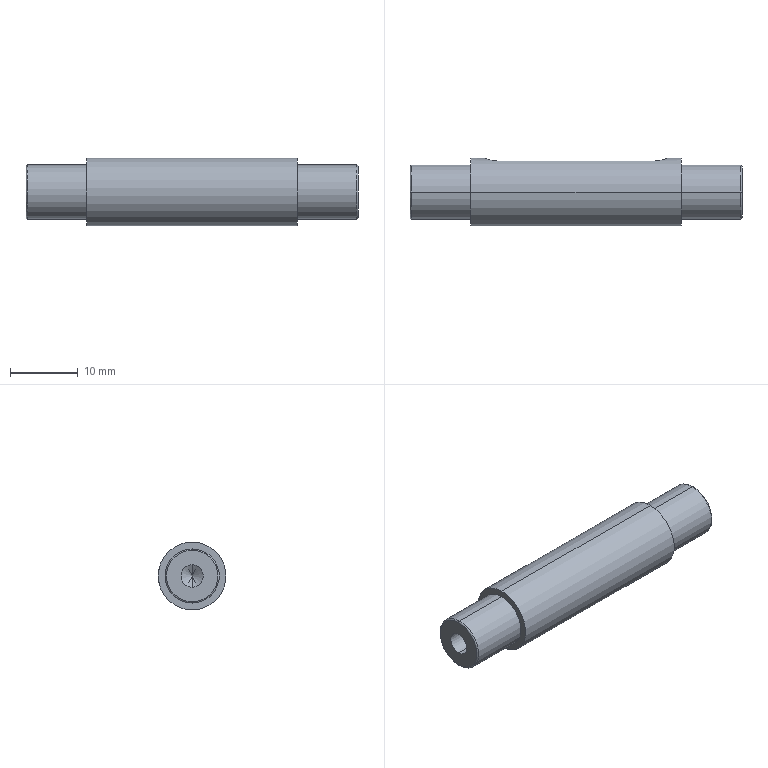Component | SolidWorks | ZHDJ-G005-1 | 1 solid | 27 faces | box 49 x 10 x 10 mm | volume 2868 mm3 | cylinder 12 | plane 7 | torus 4 | cone 4 | commonest cylinder face diameters 3.3 x4 8 x4 10 x2 4 x2
build123d program:
from build123d import *

# Parameters (mm, degrees)
SKETCH1_R                       = 5
BOSS_EXTRUDE1_DEPTH             = 15.5
CUT_EXTRUDE1_DEPTH              = 10
SKETCH4_R                       = 4
BOSS_EXTRUDE2_DEPTH             = 9
BOSS_EXTRUDE3_START             = 9
SKETCH5_R                       = 4
BOSS_EXTRUDE3_DEPTH             = 9
M4_TAPPED_HOLE1_D               = 3.3
M4_TAPPED_HOLE1_DEPTH           = 11.5
M4_TAPPED_HOLE1_TIP             = 0.9914
M4_TAPPED_HOLE1_ON_FACE_2_D     = 3.3
M4_TAPPED_HOLE1_ON_FACE_2_DEPTH = 11.5
M4_TAPPED_HOLE1_ON_FACE_2_TIP   = 0.9914
FILLET1_R                       = 0.2


with BuildPart() as part:
    # Sketch1 → Boss-Extrude1 (new, symmetric)
    with BuildSketch(Plane(origin=(0, 0, 0), x_dir=(0, 0, -1), z_dir=(1, 0, 0))):
        Circle(SKETCH1_R)
    extrude(amount=BOSS_EXTRUDE1_DEPTH, both=True)

    # Sketch3 → Cut-Extrude1 (cut)
    with BuildSketch(Plane(origin=(0, 2.3, 0), x_dir=(1, 0, 0), z_dir=(0, 1, 0))):
        with BuildLine():
            Line((11.5, -2), (-11.5, -2))
            ThreePointArc((-11.5, -2), (-13.5, 0), (-11.5, 2))
            Line((-11.5, 2), (11.5, 2))
            ThreePointArc((11.5, 2), (13.5, 0), (11.5, -2))
        make_face()
    extrude(amount=CUT_EXTRUDE1_DEPTH, mode=Mode.SUBTRACT)

    # Sketch4 → Boss-Extrude2 (add)
    with BuildSketch(Plane.ZY.offset(15.5)):
        with Locations(Location((0, 0, 0), (0, 0, 180))):
            Circle(SKETCH4_R)
    extrude(amount=BOSS_EXTRUDE2_DEPTH)

    # Sketch5 → Boss-Extrude3 (add)
    with BuildSketch(Plane(origin=(15.5, 0, 0), x_dir=(0, 0, -1), z_dir=(1, 0, 0)).offset(BOSS_EXTRUDE3_START)):
        Circle(SKETCH5_R)
    extrude(amount=-BOSS_EXTRUDE3_DEPTH)

    # M4 Tapped Hole1
    with Locations(Plane(origin=(-24.5, 0, 0), x_dir=(0, 0, -1), z_dir=(-1, 0, 0))):
        with Locations((0, 0)):
            Hole(M4_TAPPED_HOLE1_D / 2, depth=M4_TAPPED_HOLE1_DEPTH)
            with Locations((0, 0, -(M4_TAPPED_HOLE1_DEPTH + M4_TAPPED_HOLE1_TIP / 2))):  # 118° drill point
                Cone(0, M4_TAPPED_HOLE1_D / 2, M4_TAPPED_HOLE1_TIP, mode=Mode.SUBTRACT)

    # M4 Tapped Hole1 on face 2
    with Locations(Plane(origin=(24.5, 0, 0), x_dir=(0, 0, 1), z_dir=(1, 0, 0))):
        with Locations((0, 0)):
            Hole(M4_TAPPED_HOLE1_ON_FACE_2_D / 2, depth=M4_TAPPED_HOLE1_ON_FACE_2_DEPTH)
            with Locations((0, 0, -(M4_TAPPED_HOLE1_ON_FACE_2_DEPTH + M4_TAPPED_HOLE1_ON_FACE_2_TIP / 2))):  # 118° drill point
                Cone(0, M4_TAPPED_HOLE1_ON_FACE_2_D / 2, M4_TAPPED_HOLE1_ON_FACE_2_TIP, mode=Mode.SUBTRACT)

    # Fillet1
    fillet1_edges = [part.edges().sort_by_distance(p)[0] for p in [
        (-24.5, 0, 4),
        (24.5, 0, 4),
    ]]
    fillet(fillet1_edges, radius=FILLET1_R)


solid = part.part

# Placed as in the assembly
solid = solid.moved(Location((20.5, 0, -150), (0, 0, 0)))
STEP:
#1=CARTESIAN_POINT('',(1.764,0.,-5.748));
#2=VERTEX_POINT('',#1);
#3=CARTESIAN_POINT('',(1.764,0.,-6.063));
#4=VERTEX_POINT('',#3);
#5=CARTESIAN_POINT('',(1.764,0.,-5.906));
#6=DIRECTION('',(-1.,0.,0.));
#7=DIRECTION('',(0.,0.,-1.));
#8=AXIS2_PLACEMENT_3D('',#5,#6,#7);
#9=CIRCLE('',#8,0.1575);
#10=EDGE_CURVE('',#2,#4,#9,.T.);
#11=ORIENTED_EDGE('',*,*,#10,.F.);
#12=CARTESIAN_POINT('',(1.772,0.,-5.756));
#13=VERTEX_POINT('',#12);
#14=CARTESIAN_POINT('',(1.764,0.,-5.756));
#15=DIRECTION('',(0.,1.,-0.));
#16=DIRECTION('',(0.,0.,1.));
#17=AXIS2_PLACEMENT_3D('',#14,#15,#16);
#18=CIRCLE('',#17,0.007874);
#19=EDGE_CURVE('',#2,#13,#18,.T.);
#20=ORIENTED_EDGE('',*,*,#19,.T.);
#21=CARTESIAN_POINT('',(1.772,0.,-6.055));
#22=VERTEX_POINT('',#21);
#23=CARTESIAN_POINT('',(1.772,0.,-5.906));
#24=DIRECTION('',(1.,0.,0.));
#25=DIRECTION('',(0.,0.,-1.));
#26=AXIS2_PLACEMENT_3D('',#23,#24,#25);
#27=CIRCLE('',#26,0.1496);
#28=EDGE_CURVE('',#22,#13,#27,.T.);
#29=ORIENTED_EDGE('',*,*,#28,.F.);
#30=CARTESIAN_POINT('',(1.764,0.,-6.055));
#31=DIRECTION('',(0.,-1.,0.));
#32=DIRECTION('',(0.,0.,-1.));
#33=AXIS2_PLACEMENT_3D('',#30,#31,#32);
#34=CIRCLE('',#33,0.007874);
#35=EDGE_CURVE('',#4,#22,#34,.T.);
#36=ORIENTED_EDGE('',*,*,#35,.F.);
#37=EDGE_LOOP('',(#11,#20,#29,#36));
#38=FACE_OUTER_BOUND('',#37,.T.);
#39=CARTESIAN_POINT('',(1.764,0.,-5.906));
#40=DIRECTION('',(1.,0.,0.));
#41=DIRECTION('',(0.,0.,-1.));
#42=AXIS2_PLACEMENT_3D('',#39,#40,#41);
#43=TOROIDAL_SURFACE('',#42,0.1496,0.007874);
#44=ADVANCED_FACE('',(#38),#43,.T.);
#45=CARTESIAN_POINT('',(-0.1496,0.,-6.063));
#46=VERTEX_POINT('',#45);
#47=CARTESIAN_POINT('',(-0.1496,0.,-5.748));
#48=VERTEX_POINT('',#47);
#49=CARTESIAN_POINT('',(-0.1496,0.,-5.906));
#50=DIRECTION('',(1.,0.,0.));
#51=DIRECTION('',(0.,0.,1.));
#52=AXIS2_PLACEMENT_3D('',#49,#50,#51);
#53=CIRCLE('',#52,0.1575);
#54=EDGE_CURVE('',#46,#48,#53,.T.);
#55=ORIENTED_EDGE('',*,*,#54,.F.);
#56=CARTESIAN_POINT('',(-0.1575,0.,-6.055));
#57=VERTEX_POINT('',#56);
#58=CARTESIAN_POINT('',(-0.1496,0.,-6.055));
#59=DIRECTION('',(0.,1.,0.));
#60=DIRECTION('',(0.,-0.,1.));
#61=AXIS2_PLACEMENT_3D('',#58,#59,#60);
#62=CIRCLE('',#61,0.007874);
#63=EDGE_CURVE('',#46,#57,#62,.T.);
#64=ORIENTED_EDGE('',*,*,#63,.T.);
#65=CARTESIAN_POINT('',(-0.1575,0.,-5.756));
#66=VERTEX_POINT('',#65);
#67=CARTESIAN_POINT('',(-0.1575,0.,-5.906));
#68=DIRECTION('',(-1.,0.,0.));
#69=DIRECTION('',(0.,0.,1.));
#70=AXIS2_PLACEMENT_3D('',#67,#68,#69);
#71=CIRCLE('',#70,0.1496);
#72=EDGE_CURVE('',#66,#57,#71,.T.);
#73=ORIENTED_EDGE('',*,*,#72,.F.);
#74=CARTESIAN_POINT('',(-0.1496,0.,-5.756));
#75=DIRECTION('',(0.,-1.,0.));
#76=DIRECTION('',(0.,0.,-1.));
#77=AXIS2_PLACEMENT_3D('',#74,#75,#76);
#78=CIRCLE('',#77,0.007874);
#79=EDGE_CURVE('',#48,#66,#78,.T.);
#80=ORIENTED_EDGE('',*,*,#79,.F.);
#81=EDGE_LOOP('',(#55,#64,#73,#80));
#82=FACE_OUTER_BOUND('',#81,.T.);
#83=CARTESIAN_POINT('',(-0.1496,0.,-5.906));
#84=DIRECTION('',(-1.,0.,0.));
#85=DIRECTION('',(0.,0.,1.));
#86=AXIS2_PLACEMENT_3D('',#83,#84,#85);
#87=TOROIDAL_SURFACE('',#86,0.1496,0.007874);
#88=ADVANCED_FACE('',(#82),#87,.T.);
#89=CARTESIAN_POINT('',(0.2953,0.,-5.97));
#90=VERTEX_POINT('',#89);
#91=CARTESIAN_POINT('',(0.2953,0.,-5.841));
#92=VERTEX_POINT('',#91);
#93=CARTESIAN_POINT('',(0.2953,0.,-5.906));
#94=DIRECTION('',(-1.,0.,0.));
#95=DIRECTION('',(0.,0.,1.));
#96=AXIS2_PLACEMENT_3D('',#93,#94,#95);
#97=CIRCLE('',#96,0.06496);
#98=EDGE_CURVE('',#90,#92,#97,.T.);
#99=ORIENTED_EDGE('',*,*,#98,.F.);
#100=CARTESIAN_POINT('',(-0.1575,0.,-5.97));
#101=VERTEX_POINT('',#100);
#102=CARTESIAN_POINT('',(-0.1575,0.,-5.97));
#103=DIRECTION('',(-1.,0.,0.));
#104=VECTOR('',#103,39.37);
#105=LINE('',#102,#104);
#106=EDGE_CURVE('',#90,#101,#105,.T.);
#107=ORIENTED_EDGE('',*,*,#106,.T.);
#108=CARTESIAN_POINT('',(-0.1575,0.,-5.841));
#109=VERTEX_POINT('',#108);
#110=CARTESIAN_POINT('',(-0.1575,0.,-5.906));
#111=DIRECTION('',(-1.,0.,0.));
#112=DIRECTION('',(0.,0.,1.));
#113=AXIS2_PLACEMENT_3D('',#110,#111,#112);
#114=CIRCLE('',#113,0.06496);
#115=EDGE_CURVE('',#101,#109,#114,.T.);
#116=ORIENTED_EDGE('',*,*,#115,.T.);
#117=CARTESIAN_POINT('',(-0.1575,0.,-5.841));
#118=DIRECTION('',(-1.,0.,0.));
#119=VECTOR('',#118,39.37);
#120=LINE('',#117,#119);
#121=EDGE_CURVE('',#92,#109,#120,.T.);
#122=ORIENTED_EDGE('',*,*,#121,.F.);
#123=EDGE_LOOP('',(#99,#107,#116,#122));
#124=FACE_OUTER_BOUND('',#123,.T.);
#125=CARTESIAN_POINT('',(-0.1575,0.,-5.906));
#126=DIRECTION('',(-1.,0.,0.));
#127=DIRECTION('',(0.,0.,1.));
#128=AXIS2_PLACEMENT_3D('',#125,#126,#127);
#129=CYLINDRICAL_SURFACE('',#128,0.06496);
#130=ADVANCED_FACE('',(#124),#129,.F.);
#131=CARTESIAN_POINT('',(0.3343,0.,-5.906));
#132=VERTEX_POINT('',#131);
#133=CARTESIAN_POINT('',(0.2953,0.,-5.841));
#134=DIRECTION('',(-0.515,0.,0.8572));
#135=VECTOR('',#134,39.37);
#136=LINE('',#133,#135);
#137=EDGE_CURVE('',#132,#92,#136,.T.);
#138=ORIENTED_EDGE('',*,*,#137,.F.);
#139=CARTESIAN_POINT('',(0.2953,0.,-5.97));
#140=DIRECTION('',(-0.515,0.,-0.8572));
#141=VECTOR('',#140,39.37);
#142=LINE('',#139,#141);
#143=EDGE_CURVE('',#132,#90,#142,.T.);
#144=ORIENTED_EDGE('',*,*,#143,.T.);
#145=ORIENTED_EDGE('',*,*,#98,.T.);
#146=EDGE_LOOP('',(#138,#144,#145));
#147=FACE_OUTER_BOUND('',#146,.T.);
#148=CARTESIAN_POINT('',(0.2953,0.,-5.906));
#149=DIRECTION('',(-1.,0.,0.));
#150=DIRECTION('',(0.,0.,1.));
#151=AXIS2_PLACEMENT_3D('',#148,#149,#150);
#152=CONICAL_SURFACE('',#151,0.06496,1.03);
#153=ADVANCED_FACE('',(#147),#152,.F.);
#154=CARTESIAN_POINT('',(1.319,0.,-5.841));
#155=VERTEX_POINT('',#154);
#156=CARTESIAN_POINT('',(1.319,0.,-5.97));
#157=VERTEX_POINT('',#156);
#158=CARTESIAN_POINT('',(1.319,0.,-5.906));
#159=DIRECTION('',(1.,0.,0.));
#160=DIRECTION('',(0.,0.,-1.));
#161=AXIS2_PLACEMENT_3D('',#158,#159,#160);
#162=CIRCLE('',#161,0.06496);
#163=EDGE_CURVE('',#155,#157,#162,.T.);
#164=ORIENTED_EDGE('',*,*,#163,.F.);
#165=CARTESIAN_POINT('',(1.772,0.,-5.841));
#166=VERTEX_POINT('',#165);
#167=CARTESIAN_POINT('',(1.772,0.,-5.841));
#168=DIRECTION('',(1.,0.,0.));
#169=VECTOR('',#168,39.37);
#170=LINE('',#167,#169);
#171=EDGE_CURVE('',#155,#166,#170,.T.);
#172=ORIENTED_EDGE('',*,*,#171,.T.);
#173=CARTESIAN_POINT('',(1.772,0.,-5.97));
#174=VERTEX_POINT('',#173);
#175=CARTESIAN_POINT('',(1.772,0.,-5.906));
#176=DIRECTION('',(1.,0.,0.));
#177=DIRECTION('',(0.,0.,-1.));
#178=AXIS2_PLACEMENT_3D('',#175,#176,#177);
#179=CIRCLE('',#178,0.06496);
#180=EDGE_CURVE('',#166,#174,#179,.T.);
#181=ORIENTED_EDGE('',*,*,#180,.T.);
#182=CARTESIAN_POINT('',(1.772,0.,-5.97));
#183=DIRECTION('',(1.,0.,0.));
#184=VECTOR('',#183,39.37);
#185=LINE('',#182,#184);
#186=EDGE_CURVE('',#157,#174,#185,.T.);
#187=ORIENTED_EDGE('',*,*,#186,.F.);
#188=EDGE_LOOP('',(#164,#172,#181,#187));
#189=FACE_OUTER_BOUND('',#188,.T.);
#190=CARTESIAN_POINT('',(1.772,0.,-5.906));
#191=DIRECTION('',(1.,0.,0.));
#192=DIRECTION('',(0.,0.,-1.));
#193=AXIS2_PLACEMENT_3D('',#190,#191,#192);
#194=CYLINDRICAL_SURFACE('',#193,0.06496);
#195=ADVANCED_FACE('',(#189),#194,.F.);
#196=CARTESIAN_POINT('',(1.28,0.,-5.906));
#197=VERTEX_POINT('',#196);
#198=CARTESIAN_POINT('',(1.319,0.,-5.97));
#199=DIRECTION('',(0.515,0.,-0.8572));
#200=VECTOR('',#199,39.37);
#201=LINE('',#198,#200);
#202=EDGE_CURVE('',#197,#157,#201,.T.);
#203=ORIENTED_EDGE('',*,*,#202,.F.);
#204=CARTESIAN_POINT('',(1.319,0.,-5.841));
#205=DIRECTION('',(0.515,0.,0.8572));
#206=VECTOR('',#205,39.37);
#207=LINE('',#204,#206);
#208=EDGE_CURVE('',#197,#155,#207,.T.);
#209=ORIENTED_EDGE('',*,*,#208,.T.);
#210=ORIENTED_EDGE('',*,*,#163,.T.);
#211=EDGE_LOOP('',(#203,#209,#210));
#212=FACE_OUTER_BOUND('',#211,.T.);
#213=CARTESIAN_POINT('',(1.319,0.,-5.906));
#214=DIRECTION('',(1.,0.,0.));
#215=DIRECTION('',(0.,0.,-1.));
#216=AXIS2_PLACEMENT_3D('',#213,#214,#215);
#217=CONICAL_SURFACE('',#216,0.06496,1.03);
#218=ADVANCED_FACE('',(#212),#217,.F.);
#219=ORIENTED_EDGE('',*,*,#10,.T.);
#220=CARTESIAN_POINT('',(1.417,0.,-6.063));
#221=VERTEX_POINT('',#220);
#222=CARTESIAN_POINT('',(1.772,0.,-6.063));
#223=DIRECTION('',(-1.,0.,0.));
#224=VECTOR('',#223,39.37);
#225=LINE('',#222,#224);
#226=EDGE_CURVE('',#4,#221,#225,.T.);
#227=ORIENTED_EDGE('',*,*,#226,.T.);
#228=CARTESIAN_POINT('',(1.417,0.,-5.748));
#229=VERTEX_POINT('',#228);
#230=CARTESIAN_POINT('',(1.417,0.,-5.906));
#231=DIRECTION('',(1.,0.,0.));
#232=DIRECTION('',(0.,0.,-1.));
#233=AXIS2_PLACEMENT_3D('',#230,#231,#232);
#234=CIRCLE('',#233,0.1575);
#235=EDGE_CURVE('',#221,#229,#234,.T.);
#236=ORIENTED_EDGE('',*,*,#235,.T.);
#237=CARTESIAN_POINT('',(1.772,0.,-5.748));
#238=DIRECTION('',(-1.,0.,0.));
#239=VECTOR('',#238,39.37);
#240=LINE('',#237,#239);
#241=EDGE_CURVE('',#2,#229,#240,.T.);
#242=ORIENTED_EDGE('',*,*,#241,.F.);
#243=EDGE_LOOP('',(#219,#227,#236,#242));
#244=FACE_OUTER_BOUND('',#243,.T.);
#245=CARTESIAN_POINT('',(1.772,0.,-5.906));
#246=DIRECTION('',(-1.,0.,0.));
#247=DIRECTION('',(0.,0.,1.));
#248=AXIS2_PLACEMENT_3D('',#245,#246,#247);
#249=CYLINDRICAL_SURFACE('',#248,0.1575);
#250=ADVANCED_FACE('',(#244),#249,.T.);
#251=ORIENTED_EDGE('',*,*,#54,.T.);
#252=CARTESIAN_POINT('',(0.1969,0.,-5.748));
#253=VERTEX_POINT('',#252);
#254=CARTESIAN_POINT('',(-0.1575,0.,-5.748));
#255=DIRECTION('',(1.,0.,0.));
#256=VECTOR('',#255,39.37);
#257=LINE('',#254,#256);
#258=EDGE_CURVE('',#48,#253,#257,.T.);
#259=ORIENTED_EDGE('',*,*,#258,.T.);
#260=CARTESIAN_POINT('',(0.1969,0.,-6.063));
#261=VERTEX_POINT('',#260);
#262=CARTESIAN_POINT('',(0.1969,0.,-5.906));
#263=DIRECTION('',(-1.,0.,0.));
#264=DIRECTION('',(0.,0.,-1.));
#265=AXIS2_PLACEMENT_3D('',#262,#263,#264);
#266=CIRCLE('',#265,0.1575);
#267=EDGE_CURVE('',#253,#261,#266,.T.);
#268=ORIENTED_EDGE('',*,*,#267,.T.);
#269=CARTESIAN_POINT('',(-0.1575,0.,-6.063));
#270=DIRECTION('',(1.,0.,0.));
#271=VECTOR('',#270,39.37);
#272=LINE('',#269,#271);
#273=EDGE_CURVE('',#46,#261,#272,.T.);
#274=ORIENTED_EDGE('',*,*,#273,.F.);
#275=EDGE_LOOP('',(#251,#259,#268,#274));
#276=FACE_OUTER_BOUND('',#275,.T.);
#277=CARTESIAN_POINT('',(-0.1575,0.,-5.906));
#278=DIRECTION('',(1.,0.,0.));
#279=DIRECTION('',(0.,0.,-1.));
#280=AXIS2_PLACEMENT_3D('',#277,#278,#279);
#281=CYLINDRICAL_SURFACE('',#280,0.1575);
#282=ADVANCED_FACE('',(#276),#281,.T.);
#283=CARTESIAN_POINT('',(1.26,0.1804,-5.827));
#284=VERTEX_POINT('',#283);
#285=CARTESIAN_POINT('',(1.26,0.1804,-5.984));
#286=VERTEX_POINT('',#285);
#287=CARTESIAN_POINT('',(1.26,0.1804,-5.827));
#288=CARTESIAN_POINT('',(1.265,0.1804,-5.827));
#289=CARTESIAN_POINT('',(1.27,0.1806,-5.827));
#290=CARTESIAN_POINT('',(1.28,0.1815,-5.829));
#291=CARTESIAN_POINT('',(1.285,0.1822,-5.831));
#292=CARTESIAN_POINT('',(1.295,0.1837,-5.835));
#293=CARTESIAN_POINT('',(1.299,0.1847,-5.837));
#294=CARTESIAN_POINT('',(1.308,0.1867,-5.843));
#295=CARTESIAN_POINT('',(1.312,0.1877,-5.846));
#296=CARTESIAN_POINT('',(1.323,0.1909,-5.857));
#297=CARTESIAN_POINT('',(1.329,0.193,-5.866));
#298=CARTESIAN_POINT('',(1.334,0.1952,-5.88));
#299=CARTESIAN_POINT('',(1.336,0.1958,-5.885));
#300=CARTESIAN_POINT('',(1.338,0.1966,-5.895));
#301=CARTESIAN_POINT('',(1.339,0.1968,-5.9));
#302=CARTESIAN_POINT('',(1.339,0.1969,-5.911));
#303=CARTESIAN_POINT('',(1.338,0.1966,-5.916));
#304=CARTESIAN_POINT('',(1.336,0.1958,-5.926));
#305=CARTESIAN_POINT('',(1.335,0.1953,-5.931));
#306=CARTESIAN_POINT('',(1.331,0.1938,-5.941));
#307=CARTESIAN_POINT('',(1.328,0.1929,-5.945));
#308=CARTESIAN_POINT('',(1.322,0.1909,-5.954));
#309=CARTESIAN_POINT('',(1.319,0.1899,-5.958));
#310=CARTESIAN_POINT('',(1.312,0.1878,-5.965));
#311=CARTESIAN_POINT('',(1.308,0.1867,-5.968));
#312=CARTESIAN_POINT('',(1.3,0.1847,-5.974));
#313=CARTESIAN_POINT('',(1.295,0.1837,-5.976));
#314=CARTESIAN_POINT('',(1.281,0.1814,-5.982));
#315=CARTESIAN_POINT('',(1.27,0.1804,-5.984));
#316=CARTESIAN_POINT('',(1.26,0.1804,-5.984));
#317=B_SPLINE_CURVE_WITH_KNOTS('',3,(#287,#288,#289,#290,#291,#292,#293,#294,#295,#296,#297,#298,#299,#300,#301,#302,#303,#304,#305,#306,#307,#308,#309,#310,#311,#312,#313,#314,#315,#316),.UNSPECIFIED.,.F.,.F.,(4,2,2,2,2,2,2,2,2,2,2,2,2,2,4),(0.,0.0003948,0.0007896,0.001184,0.001579,0.002369,0.002764,0.003158,0.003553,0.003948,0.004343,0.004737,0.005132,0.005527,0.006317),.UNSPECIFIED.);
#318=EDGE_CURVE('',#284,#286,#317,.T.);
#319=ORIENTED_EDGE('',*,*,#318,.F.);
#320=CARTESIAN_POINT('',(0.3543,0.1804,-5.827));
#321=VERTEX_POINT('',#320);
#322=CARTESIAN_POINT('',(1.417,0.1804,-5.827));
#323=DIRECTION('',(1.,0.,0.));
#324=VECTOR('',#323,39.37);
#325=LINE('',#322,#324);
#326=EDGE_CURVE('',#321,#284,#325,.T.);
#327=ORIENTED_EDGE('',*,*,#326,.F.);
#328=CARTESIAN_POINT('',(0.3543,0.1804,-5.984));
#329=VERTEX_POINT('',#328);
#330=CARTESIAN_POINT('',(0.3543,0.1804,-5.984));
#331=CARTESIAN_POINT('',(0.3491,0.1804,-5.984));
#332=CARTESIAN_POINT('',(0.3439,0.1806,-5.984));
#333=CARTESIAN_POINT('',(0.3338,0.1815,-5.982));
#334=CARTESIAN_POINT('',(0.3288,0.1822,-5.98));
#335=CARTESIAN_POINT('',(0.3193,0.1837,-5.976));
#336=CARTESIAN_POINT('',(0.3148,0.1847,-5.974));
#337=CARTESIAN_POINT('',(0.3062,0.1867,-5.968));
#338=CARTESIAN_POINT('',(0.3023,0.1877,-5.965));
#339=CARTESIAN_POINT('',(0.2915,0.1909,-5.954));
#340=CARTESIAN_POINT('',(0.2856,0.193,-5.945));
#341=CARTESIAN_POINT('',(0.2797,0.1952,-5.931));
#342=CARTESIAN_POINT('',(0.2782,0.1958,-5.926));
#343=CARTESIAN_POINT('',(0.2761,0.1966,-5.916));
#344=CARTESIAN_POINT('',(0.2756,0.1968,-5.911));
#345=CARTESIAN_POINT('',(0.2756,0.1969,-5.9));
#346=CARTESIAN_POINT('',(0.2761,0.1966,-5.895));
#347=CARTESIAN_POINT('',(0.2781,0.1958,-5.885));
#348=CARTESIAN_POINT('',(0.2796,0.1953,-5.88));
#349=CARTESIAN_POINT('',(0.2836,0.1938,-5.87));
#350=CARTESIAN_POINT('',(0.2861,0.1929,-5.866));
#351=CARTESIAN_POINT('',(0.2918,0.1909,-5.857));
#352=CARTESIAN_POINT('',(0.295,0.1899,-5.853));
#353=CARTESIAN_POINT('',(0.3023,0.1878,-5.846));
#354=CARTESIAN_POINT('',(0.3062,0.1867,-5.843));
#355=CARTESIAN_POINT('',(0.3147,0.1847,-5.837));
#356=CARTESIAN_POINT('',(0.3192,0.1837,-5.835));
#357=CARTESIAN_POINT('',(0.3334,0.1814,-5.829));
#358=CARTESIAN_POINT('',(0.3438,0.1804,-5.827));
#359=CARTESIAN_POINT('',(0.3543,0.1804,-5.827));
#360=B_SPLINE_CURVE_WITH_KNOTS('',3,(#330,#331,#332,#333,#334,#335,#336,#337,#338,#339,#340,#341,#342,#343,#344,#345,#346,#347,#348,#349,#350,#351,#352,#353,#354,#355,#356,#357,#358,#359),.UNSPECIFIED.,.F.,.F.,(4,2,2,2,2,2,2,2,2,2,2,2,2,2,4),(0.,0.0003948,0.0007896,0.001184,0.001579,0.002369,0.002764,0.003158,0.003553,0.003948,0.004343,0.004737,0.005132,0.005527,0.006317),.UNSPECIFIED.);
#361=EDGE_CURVE('',#329,#321,#360,.T.);
#362=ORIENTED_EDGE('',*,*,#361,.F.);
#363=CARTESIAN_POINT('',(1.417,0.1804,-5.984));
#364=DIRECTION('',(-1.,0.,0.));
#365=VECTOR('',#364,39.37);
#366=LINE('',#363,#365);
#367=EDGE_CURVE('',#286,#329,#366,.T.);
#368=ORIENTED_EDGE('',*,*,#367,.F.);
#369=EDGE_LOOP('',(#319,#327,#362,#368));
#370=FACE_BOUND('',#369,.T.);
#371=CARTESIAN_POINT('',(1.417,0.,-6.102));
#372=VERTEX_POINT('',#371);
#373=CARTESIAN_POINT('',(1.417,0.,-5.709));
#374=VERTEX_POINT('',#373);
#375=CARTESIAN_POINT('',(1.417,0.,-5.906));
#376=DIRECTION('',(1.,0.,0.));
#377=DIRECTION('',(0.,0.,-1.));
#378=AXIS2_PLACEMENT_3D('',#375,#376,#377);
#379=CIRCLE('',#378,0.1969);
#380=EDGE_CURVE('',#372,#374,#379,.T.);
#381=ORIENTED_EDGE('',*,*,#380,.F.);
#382=CARTESIAN_POINT('',(0.1969,0.,-6.102));
#383=VERTEX_POINT('',#382);
#384=CARTESIAN_POINT('',(1.417,0.,-6.102));
#385=DIRECTION('',(-1.,0.,0.));
#386=VECTOR('',#385,39.37);
#387=LINE('',#384,#386);
#388=EDGE_CURVE('',#372,#383,#387,.T.);
#389=ORIENTED_EDGE('',*,*,#388,.T.);
#390=CARTESIAN_POINT('',(0.1969,0.,-5.709));
#391=VERTEX_POINT('',#390);
#392=CARTESIAN_POINT('',(0.1969,0.,-5.906));
#393=DIRECTION('',(1.,0.,0.));
#394=DIRECTION('',(0.,0.,-1.));
#395=AXIS2_PLACEMENT_3D('',#392,#393,#394);
#396=CIRCLE('',#395,0.1969);
#397=EDGE_CURVE('',#383,#391,#396,.T.);
#398=ORIENTED_EDGE('',*,*,#397,.T.);
#399=CARTESIAN_POINT('',(1.417,0.,-5.709));
#400=DIRECTION('',(-1.,0.,0.));
#401=VECTOR('',#400,39.37);
#402=LINE('',#399,#401);
#403=EDGE_CURVE('',#374,#391,#402,.T.);
#404=ORIENTED_EDGE('',*,*,#403,.F.);
#405=EDGE_LOOP('',(#381,#389,#398,#404));
#406=FACE_OUTER_BOUND('',#405,.T.);
#407=CARTESIAN_POINT('',(1.417,0.,-5.906));
#408=DIRECTION('',(-1.,0.,0.));
#409=DIRECTION('',(0.,0.,1.));
#410=AXIS2_PLACEMENT_3D('',#407,#408,#409);
#411=CYLINDRICAL_SURFACE('',#410,0.1969);
#412=ADVANCED_FACE('',(#370,#406),#411,.T.);
#413=ORIENTED_EDGE('',*,*,#388,.F.);
#414=CARTESIAN_POINT('',(1.417,0.,-5.906));
#415=DIRECTION('',(1.,0.,0.));
#416=DIRECTION('',(0.,0.,-1.));
#417=AXIS2_PLACEMENT_3D('',#414,#415,#416);
#418=CIRCLE('',#417,0.1969);
#419=EDGE_CURVE('',#374,#372,#418,.T.);
#420=ORIENTED_EDGE('',*,*,#419,.F.);
#421=ORIENTED_EDGE('',*,*,#403,.T.);
#422=CARTESIAN_POINT('',(0.1969,0.,-5.906));
#423=DIRECTION('',(1.,0.,0.));
#424=DIRECTION('',(0.,0.,-1.));
#425=AXIS2_PLACEMENT_3D('',#422,#423,#424);
#426=CIRCLE('',#425,0.1969);
#427=EDGE_CURVE('',#391,#383,#426,.T.);
#428=ORIENTED_EDGE('',*,*,#427,.T.);
#429=EDGE_LOOP('',(#413,#420,#421,#428));
#430=FACE_OUTER_BOUND('',#429,.T.);
#431=CARTESIAN_POINT('',(1.417,0.,-5.906));
#432=DIRECTION('',(-1.,0.,0.));
#433=DIRECTION('',(0.,0.,1.));
#434=AXIS2_PLACEMENT_3D('',#431,#432,#433);
#435=CYLINDRICAL_SURFACE('',#434,0.1969);
#436=ADVANCED_FACE('',(#430),#435,.T.);
#437=CARTESIAN_POINT('',(1.417,0.,-5.906));
#438=DIRECTION('',(1.,0.,0.));
#439=DIRECTION('',(0.,0.,-1.));
#440=AXIS2_PLACEMENT_3D('',#437,#438,#439);
#441=CIRCLE('',#440,0.1575);
#442=EDGE_CURVE('',#229,#221,#441,.T.);
#443=ORIENTED_EDGE('',*,*,#442,.F.);
#444=ORIENTED_EDGE('',*,*,#235,.F.);
#445=EDGE_LOOP('',(#443,#444));
#446=FACE_BOUND('',#445,.T.);
#447=ORIENTED_EDGE('',*,*,#419,.T.);
#448=ORIENTED_EDGE('',*,*,#380,.T.);
#449=EDGE_LOOP('',(#447,#448));
#450=FACE_OUTER_BOUND('',#449,.T.);
#451=CARTESIAN_POINT('',(1.417,0.,-5.906));
#452=DIRECTION('',(1.,0.,0.));
#453=DIRECTION('',(0.,0.,-1.));
#454=AXIS2_PLACEMENT_3D('',#451,#452,#453);
#455=PLANE('',#454);
#456=ADVANCED_FACE('',(#446,#450),#455,.T.);
#457=CARTESIAN_POINT('',(0.1969,0.,-5.906));
#458=DIRECTION('',(-1.,0.,0.));
#459=DIRECTION('',(0.,0.,-1.));
#460=AXIS2_PLACEMENT_3D('',#457,#458,#459);
#461=CIRCLE('',#460,0.1575);
#462=EDGE_CURVE('',#261,#253,#461,.T.);
#463=ORIENTED_EDGE('',*,*,#462,.F.);
#464=ORIENTED_EDGE('',*,*,#267,.F.);
#465=EDGE_LOOP('',(#463,#464));
#466=FACE_BOUND('',#465,.T.);
#467=ORIENTED_EDGE('',*,*,#427,.F.);
#468=ORIENTED_EDGE('',*,*,#397,.F.);
#469=EDGE_LOOP('',(#467,#468));
#470=FACE_OUTER_BOUND('',#469,.T.);
#471=CARTESIAN_POINT('',(0.1969,0.,-5.906));
#472=DIRECTION('',(1.,0.,0.));
#473=DIRECTION('',(0.,0.,-1.));
#474=AXIS2_PLACEMENT_3D('',#471,#472,#473);
#475=PLANE('',#474);
#476=ADVANCED_FACE('',(#466,#470),#475,.F.);
#477=ORIENTED_EDGE('',*,*,#318,.T.);
#478=CARTESIAN_POINT('',(1.26,0.09055,-5.984));
#479=VERTEX_POINT('',#478);
#480=CARTESIAN_POINT('',(1.26,0.4843,-5.984));
#481=DIRECTION('',(0.,-1.,0.));
#482=VECTOR('',#481,39.37);
#483=LINE('',#480,#482);
#484=EDGE_CURVE('',#286,#479,#483,.T.);
#485=ORIENTED_EDGE('',*,*,#484,.T.);
#486=CARTESIAN_POINT('',(1.26,0.09055,-5.827));
#487=VERTEX_POINT('',#486);
#488=CARTESIAN_POINT('',(1.26,0.09055,-5.906));
#489=DIRECTION('',(0.,1.,0.));
#490=DIRECTION('',(0.,0.,1.));
#491=AXIS2_PLACEMENT_3D('',#488,#489,#490);
#492=CIRCLE('',#491,0.07874);
#493=EDGE_CURVE('',#487,#479,#492,.T.);
#494=ORIENTED_EDGE('',*,*,#493,.F.);
#495=CARTESIAN_POINT('',(1.26,0.4843,-5.827));
#496=DIRECTION('',(0.,-1.,0.));
#497=VECTOR('',#496,39.37);
#498=LINE('',#495,#497);
#499=EDGE_CURVE('',#284,#487,#498,.T.);
#500=ORIENTED_EDGE('',*,*,#499,.F.);
#501=EDGE_LOOP('',(#477,#485,#494,#500));
#502=FACE_OUTER_BOUND('',#501,.T.);
#503=CARTESIAN_POINT('',(1.26,0.4843,-5.906));
#504=DIRECTION('',(0.,-1.,0.));
#505=DIRECTION('',(0.,0.,-1.));
#506=AXIS2_PLACEMENT_3D('',#503,#504,#505);
#507=CYLINDRICAL_SURFACE('',#506,0.07874);
#508=ADVANCED_FACE('',(#502),#507,.F.);
#509=ORIENTED_EDGE('',*,*,#367,.T.);
#510=CARTESIAN_POINT('',(0.3543,0.09055,-5.984));
#511=VERTEX_POINT('',#510);
#512=CARTESIAN_POINT('',(0.3543,0.4843,-5.984));
#513=DIRECTION('',(0.,-1.,0.));
#514=VECTOR('',#513,39.37);
#515=LINE('',#512,#514);
#516=EDGE_CURVE('',#329,#511,#515,.T.);
#517=ORIENTED_EDGE('',*,*,#516,.T.);
#518=CARTESIAN_POINT('',(1.26,0.09055,-5.984));
#519=DIRECTION('',(-1.,0.,0.));
#520=VECTOR('',#519,39.37);
#521=LINE('',#518,#520);
#522=EDGE_CURVE('',#479,#511,#521,.T.);
#523=ORIENTED_EDGE('',*,*,#522,.F.);
#524=ORIENTED_EDGE('',*,*,#484,.F.);
#525=EDGE_LOOP('',(#509,#517,#523,#524));
#526=FACE_OUTER_BOUND('',#525,.T.);
#527=CARTESIAN_POINT('',(1.26,0.4843,-5.984));
#528=DIRECTION('',(0.,0.,1.));
#529=DIRECTION('',(1.,0.,-0.));
#530=AXIS2_PLACEMENT_3D('',#527,#528,#529);
#531=PLANE('',#530);
#532=ADVANCED_FACE('',(#526),#531,.T.);
#533=ORIENTED_EDGE('',*,*,#361,.T.);
#534=CARTESIAN_POINT('',(0.3543,0.09055,-5.827));
#535=VERTEX_POINT('',#534);
#536=CARTESIAN_POINT('',(0.3543,0.4843,-5.827));
#537=DIRECTION('',(0.,-1.,0.));
#538=VECTOR('',#537,39.37);
#539=LINE('',#536,#538);
#540=EDGE_CURVE('',#321,#535,#539,.T.);
#541=ORIENTED_EDGE('',*,*,#540,.T.);
#542=CARTESIAN_POINT('',(0.3543,0.09055,-5.906));
#543=DIRECTION('',(0.,1.,0.));
#544=DIRECTION('',(0.,0.,1.));
#545=AXIS2_PLACEMENT_3D('',#542,#543,#544);
#546=CIRCLE('',#545,0.07874);
#547=EDGE_CURVE('',#511,#535,#546,.T.);
#548=ORIENTED_EDGE('',*,*,#547,.F.);
#549=ORIENTED_EDGE('',*,*,#516,.F.);
#550=EDGE_LOOP('',(#533,#541,#548,#549));
#551=FACE_OUTER_BOUND('',#550,.T.);
#552=CARTESIAN_POINT('',(0.3543,0.4843,-5.906));
#553=DIRECTION('',(0.,-1.,0.));
#554=DIRECTION('',(0.,0.,-1.));
#555=AXIS2_PLACEMENT_3D('',#552,#553,#554);
#556=CYLINDRICAL_SURFACE('',#555,0.07874);
#557=ADVANCED_FACE('',(#551),#556,.F.);
#558=ORIENTED_EDGE('',*,*,#326,.T.);
#559=ORIENTED_EDGE('',*,*,#499,.T.);
#560=CARTESIAN_POINT('',(1.26,0.09055,-5.827));
#561=DIRECTION('',(1.,0.,-0.));
#562=VECTOR('',#561,39.37);
#563=LINE('',#560,#562);
#564=EDGE_CURVE('',#535,#487,#563,.T.);
#565=ORIENTED_EDGE('',*,*,#564,.F.);
#566=ORIENTED_EDGE('',*,*,#540,.F.);
#567=EDGE_LOOP('',(#558,#559,#565,#566));
#568=FACE_OUTER_BOUND('',#567,.T.);
#569=CARTESIAN_POINT('',(1.26,0.4843,-5.827));
#570=DIRECTION('',(-0.,0.,-1.));
#571=DIRECTION('',(-1.,0.,0.));
#572=AXIS2_PLACEMENT_3D('',#569,#570,#571);
#573=PLANE('',#572);
#574=ADVANCED_FACE('',(#568),#573,.T.);
#575=ORIENTED_EDGE('',*,*,#493,.T.);
#576=ORIENTED_EDGE('',*,*,#522,.T.);
#577=ORIENTED_EDGE('',*,*,#547,.T.);
#578=ORIENTED_EDGE('',*,*,#564,.T.);
#579=EDGE_LOOP('',(#575,#576,#577,#578));
#580=FACE_OUTER_BOUND('',#579,.T.);
#581=CARTESIAN_POINT('',(1.26,0.09055,-5.906));
#582=DIRECTION('',(0.,1.,0.));
#583=DIRECTION('',(0.,0.,1.));
#584=AXIS2_PLACEMENT_3D('',#581,#582,#583);
#585=PLANE('',#584);
#586=ADVANCED_FACE('',(#580),#585,.T.);
#587=ORIENTED_EDGE('',*,*,#258,.F.);
#588=CARTESIAN_POINT('',(-0.1496,0.,-5.906));
#589=DIRECTION('',(1.,0.,0.));
#590=DIRECTION('',(0.,0.,1.));
#591=AXIS2_PLACEMENT_3D('',#588,#589,#590);
#592=CIRCLE('',#591,0.1575);
#593=EDGE_CURVE('',#48,#46,#592,.T.);
#594=ORIENTED_EDGE('',*,*,#593,.T.);
#595=ORIENTED_EDGE('',*,*,#273,.T.);
#596=ORIENTED_EDGE('',*,*,#462,.T.);
#597=EDGE_LOOP('',(#587,#594,#595,#596));
#598=FACE_OUTER_BOUND('',#597,.T.);
#599=CARTESIAN_POINT('',(-0.1575,0.,-5.906));
#600=DIRECTION('',(1.,0.,0.));
#601=DIRECTION('',(0.,0.,-1.));
#602=AXIS2_PLACEMENT_3D('',#599,#600,#601);
#603=CYLINDRICAL_SURFACE('',#602,0.1575);
#604=ADVANCED_FACE('',(#598),#603,.T.);
#605=ORIENTED_EDGE('',*,*,#72,.T.);
#606=CARTESIAN_POINT('',(-0.1575,0.,-5.906));
#607=DIRECTION('',(-1.,0.,0.));
#608=DIRECTION('',(0.,0.,1.));
#609=AXIS2_PLACEMENT_3D('',#606,#607,#608);
#610=CIRCLE('',#609,0.1496);
#611=EDGE_CURVE('',#57,#66,#610,.T.);
#612=ORIENTED_EDGE('',*,*,#611,.T.);
#613=EDGE_LOOP('',(#605,#612));
#614=FACE_OUTER_BOUND('',#613,.T.);
#615=CARTESIAN_POINT('',(-0.1575,0.,-5.906));
#616=DIRECTION('',(-1.,0.,0.));
#617=DIRECTION('',(0.,0.,1.));
#618=AXIS2_PLACEMENT_3D('',#615,#616,#617);
#619=CIRCLE('',#618,0.06496);
#620=EDGE_CURVE('',#109,#101,#619,.T.);
#621=ORIENTED_EDGE('',*,*,#620,.F.);
#622=ORIENTED_EDGE('',*,*,#115,.F.);
#623=EDGE_LOOP('',(#621,#622));
#624=FACE_BOUND('',#623,.T.);
#625=CARTESIAN_POINT('',(-0.1575,0.,-5.906));
#626=DIRECTION('',(-1.,0.,0.));
#627=DIRECTION('',(0.,0.,1.));
#628=AXIS2_PLACEMENT_3D('',#625,#626,#627);
#629=PLANE('',#628);
#630=ADVANCED_FACE('',(#614,#624),#629,.T.);
#631=ORIENTED_EDGE('',*,*,#226,.F.);
#632=CARTESIAN_POINT('',(1.764,0.,-5.906));
#633=DIRECTION('',(-1.,0.,0.));
#634=DIRECTION('',(0.,0.,-1.));
#635=AXIS2_PLACEMENT_3D('',#632,#633,#634);
#636=CIRCLE('',#635,0.1575);
#637=EDGE_CURVE('',#4,#2,#636,.T.);
#638=ORIENTED_EDGE('',*,*,#637,.T.);
#639=ORIENTED_EDGE('',*,*,#241,.T.);
#640=ORIENTED_EDGE('',*,*,#442,.T.);
#641=EDGE_LOOP('',(#631,#638,#639,#640));
#642=FACE_OUTER_BOUND('',#641,.T.);
#643=CARTESIAN_POINT('',(1.772,0.,-5.906));
#644=DIRECTION('',(-1.,0.,0.));
#645=DIRECTION('',(0.,0.,1.));
#646=AXIS2_PLACEMENT_3D('',#643,#644,#645);
#647=CYLINDRICAL_SURFACE('',#646,0.1575);
#648=ADVANCED_FACE('',(#642),#647,.T.);
#649=ORIENTED_EDGE('',*,*,#28,.T.);
#650=CARTESIAN_POINT('',(1.772,0.,-5.906));
#651=DIRECTION('',(1.,0.,0.));
#652=DIRECTION('',(0.,0.,-1.));
#653=AXIS2_PLACEMENT_3D('',#650,#651,#652);
#654=CIRCLE('',#653,0.1496);
#655=EDGE_CURVE('',#13,#22,#654,.T.);
#656=ORIENTED_EDGE('',*,*,#655,.T.);
#657=EDGE_LOOP('',(#649,#656));
#658=FACE_OUTER_BOUND('',#657,.T.);
#659=CARTESIAN_POINT('',(1.772,0.,-5.906));
#660=DIRECTION('',(1.,0.,0.));
#661=DIRECTION('',(0.,0.,-1.));
#662=AXIS2_PLACEMENT_3D('',#659,#660,#661);
#663=CIRCLE('',#662,0.06496);
#664=EDGE_CURVE('',#174,#166,#663,.T.);
#665=ORIENTED_EDGE('',*,*,#664,.F.);
#666=ORIENTED_EDGE('',*,*,#180,.F.);
#667=EDGE_LOOP('',(#665,#666));
#668=FACE_BOUND('',#667,.T.);
#669=CARTESIAN_POINT('',(1.772,0.,-5.906));
#670=DIRECTION('',(1.,0.,0.));
#671=DIRECTION('',(0.,0.,-1.));
#672=AXIS2_PLACEMENT_3D('',#669,#670,#671);
#673=PLANE('',#672);
#674=ADVANCED_FACE('',(#658,#668),#673,.T.);
#675=ORIENTED_EDGE('',*,*,#208,.F.);
#676=ORIENTED_EDGE('',*,*,#202,.T.);
#677=CARTESIAN_POINT('',(1.319,0.,-5.906));
#678=DIRECTION('',(1.,0.,0.));
#679=DIRECTION('',(0.,0.,-1.));
#680=AXIS2_PLACEMENT_3D('',#677,#678,#679);
#681=CIRCLE('',#680,0.06496);
#682=EDGE_CURVE('',#157,#155,#681,.T.);
#683=ORIENTED_EDGE('',*,*,#682,.T.);
#684=EDGE_LOOP('',(#675,#676,#683));
#685=FACE_OUTER_BOUND('',#684,.T.);
#686=CARTESIAN_POINT('',(1.319,0.,-5.906));
#687=DIRECTION('',(1.,0.,0.));
#688=DIRECTION('',(0.,0.,-1.));
#689=AXIS2_PLACEMENT_3D('',#686,#687,#688);
#690=CONICAL_SURFACE('',#689,0.06496,1.03);
#691=ADVANCED_FACE('',(#685),#690,.F.);
#692=ORIENTED_EDGE('',*,*,#171,.F.);
#693=ORIENTED_EDGE('',*,*,#682,.F.);
#694=ORIENTED_EDGE('',*,*,#186,.T.);
#695=ORIENTED_EDGE('',*,*,#664,.T.);
#696=EDGE_LOOP('',(#692,#693,#694,#695));
#697=FACE_OUTER_BOUND('',#696,.T.);
#698=CARTESIAN_POINT('',(1.772,0.,-5.906));
#699=DIRECTION('',(1.,0.,0.));
#700=DIRECTION('',(0.,0.,-1.));
#701=AXIS2_PLACEMENT_3D('',#698,#699,#700);
#702=CYLINDRICAL_SURFACE('',#701,0.06496);
#703=ADVANCED_FACE('',(#697),#702,.F.);
#704=ORIENTED_EDGE('',*,*,#143,.F.);
#705=ORIENTED_EDGE('',*,*,#137,.T.);
#706=CARTESIAN_POINT('',(0.2953,0.,-5.906));
#707=DIRECTION('',(-1.,0.,0.));
#708=DIRECTION('',(0.,0.,1.));
#709=AXIS2_PLACEMENT_3D('',#706,#707,#708);
#710=CIRCLE('',#709,0.06496);
#711=EDGE_CURVE('',#92,#90,#710,.T.);
#712=ORIENTED_EDGE('',*,*,#711,.T.);
#713=EDGE_LOOP('',(#704,#705,#712));
#714=FACE_OUTER_BOUND('',#713,.T.);
#715=CARTESIAN_POINT('',(0.2953,0.,-5.906));
#716=DIRECTION('',(-1.,0.,0.));
#717=DIRECTION('',(0.,0.,1.));
#718=AXIS2_PLACEMENT_3D('',#715,#716,#717);
#719=CONICAL_SURFACE('',#718,0.06496,1.03);
#720=ADVANCED_FACE('',(#714),#719,.F.);
#721=ORIENTED_EDGE('',*,*,#106,.F.);
#722=ORIENTED_EDGE('',*,*,#711,.F.);
#723=ORIENTED_EDGE('',*,*,#121,.T.);
#724=ORIENTED_EDGE('',*,*,#620,.T.);
#725=EDGE_LOOP('',(#721,#722,#723,#724));
#726=FACE_OUTER_BOUND('',#725,.T.);
#727=CARTESIAN_POINT('',(-0.1575,0.,-5.906));
#728=DIRECTION('',(-1.,0.,0.));
#729=DIRECTION('',(0.,0.,1.));
#730=AXIS2_PLACEMENT_3D('',#727,#728,#729);
#731=CYLINDRICAL_SURFACE('',#730,0.06496);
#732=ADVANCED_FACE('',(#726),#731,.F.);
#733=ORIENTED_EDGE('',*,*,#63,.F.);
#734=ORIENTED_EDGE('',*,*,#593,.F.);
#735=ORIENTED_EDGE('',*,*,#79,.T.);
#736=ORIENTED_EDGE('',*,*,#611,.F.);
#737=EDGE_LOOP('',(#733,#734,#735,#736));
#738=FACE_OUTER_BOUND('',#737,.T.);
#739=CARTESIAN_POINT('',(-0.1496,0.,-5.906));
#740=DIRECTION('',(-1.,0.,0.));
#741=DIRECTION('',(0.,0.,1.));
#742=AXIS2_PLACEMENT_3D('',#739,#740,#741);
#743=TOROIDAL_SURFACE('',#742,0.1496,0.007874);
#744=ADVANCED_FACE('',(#738),#743,.T.);
#745=ORIENTED_EDGE('',*,*,#19,.F.);
#746=ORIENTED_EDGE('',*,*,#637,.F.);
#747=ORIENTED_EDGE('',*,*,#35,.T.);
#748=ORIENTED_EDGE('',*,*,#655,.F.);
#749=EDGE_LOOP('',(#745,#746,#747,#748));
#750=FACE_OUTER_BOUND('',#749,.T.);
#751=CARTESIAN_POINT('',(1.764,0.,-5.906));
#752=DIRECTION('',(1.,0.,0.));
#753=DIRECTION('',(0.,0.,-1.));
#754=AXIS2_PLACEMENT_3D('',#751,#752,#753);
#755=TOROIDAL_SURFACE('',#754,0.1496,0.007874);
#756=ADVANCED_FACE('',(#750),#755,.T.);
#757=CLOSED_SHELL('',(#44,#88,#130,#153,#195,#218,#250,#282,#412,#436,#456,#476,#508,#532,#557,#574,#586,#604,#630,#648,#674,#691,#703,#720,#732,#744,#756));
#758=MANIFOLD_SOLID_BREP('',#757);
#759=CARTESIAN_POINT('',(0.,0.,0.));
#760=DIRECTION('',(0.,0.,1.));
#761=DIRECTION('',(1.,0.,0.));
#762=AXIS2_PLACEMENT_3D('',#759,#760,#761);
#763=(LENGTH_UNIT()NAMED_UNIT(*)SI_UNIT($,.METRE.));
#764=LENGTH_MEASURE_WITH_UNIT(LENGTH_MEASURE(0.0254),#763);
#765=DIMENSIONAL_EXPONENTS(1.,0.,0.,0.,0.,0.,0.);
#766=(CONVERSION_BASED_UNIT('',#764)LENGTH_UNIT()NAMED_UNIT(#765));
#767=UNCERTAINTY_MEASURE_WITH_UNIT(LENGTH_MEASURE(0.00001),#766,'','');
#768=(NAMED_UNIT(*)PLANE_ANGLE_UNIT()SI_UNIT($,.RADIAN.));
#769=(NAMED_UNIT(*)SI_UNIT($,.STERADIAN.)SOLID_ANGLE_UNIT());
#770=(GEOMETRIC_REPRESENTATION_CONTEXT(3)GLOBAL_UNCERTAINTY_ASSIGNED_CONTEXT((#767))GLOBAL_UNIT_ASSIGNED_CONTEXT((#766,#768,#769))REPRESENTATION_CONTEXT('',''));
#771=ADVANCED_BREP_SHAPE_REPRESENTATION('',(#758,#762),#770);
#772=COLOUR_RGB('',0.7922,0.8196,0.9333);
#773=FILL_AREA_STYLE_COLOUR('',#772);
#774=FILL_AREA_STYLE('',(#773));
#775=SURFACE_STYLE_FILL_AREA(#774);
#776=SURFACE_SIDE_STYLE('',(#775));
#777=SURFACE_STYLE_USAGE(.BOTH.,#776);
#778=PRESENTATION_STYLE_ASSIGNMENT((#777));
#779=STYLED_ITEM('',(#778),#758);
#780=PRESENTATION_LAYER_ASSIGNMENT('','',(#779));
#781=(LENGTH_UNIT()NAMED_UNIT(*)SI_UNIT($,.METRE.));
#782=LENGTH_MEASURE_WITH_UNIT(LENGTH_MEASURE(0.0254),#781);
#783=DIMENSIONAL_EXPONENTS(1.,0.,0.,0.,0.,0.,0.);
#784=(CONVERSION_BASED_UNIT('',#782)LENGTH_UNIT()NAMED_UNIT(#783));
#785=UNCERTAINTY_MEASURE_WITH_UNIT(LENGTH_MEASURE(0.00001),#784,'','');
#786=(NAMED_UNIT(*)PLANE_ANGLE_UNIT()SI_UNIT($,.RADIAN.));
#787=(NAMED_UNIT(*)SI_UNIT($,.STERADIAN.)SOLID_ANGLE_UNIT());
#788=(GEOMETRIC_REPRESENTATION_CONTEXT(3)GLOBAL_UNCERTAINTY_ASSIGNED_CONTEXT((#785))GLOBAL_UNIT_ASSIGNED_CONTEXT((#784,#786,#787))REPRESENTATION_CONTEXT('',''));
#789=MECHANICAL_DESIGN_GEOMETRIC_PRESENTATION_REPRESENTATION('',(#779),#788);